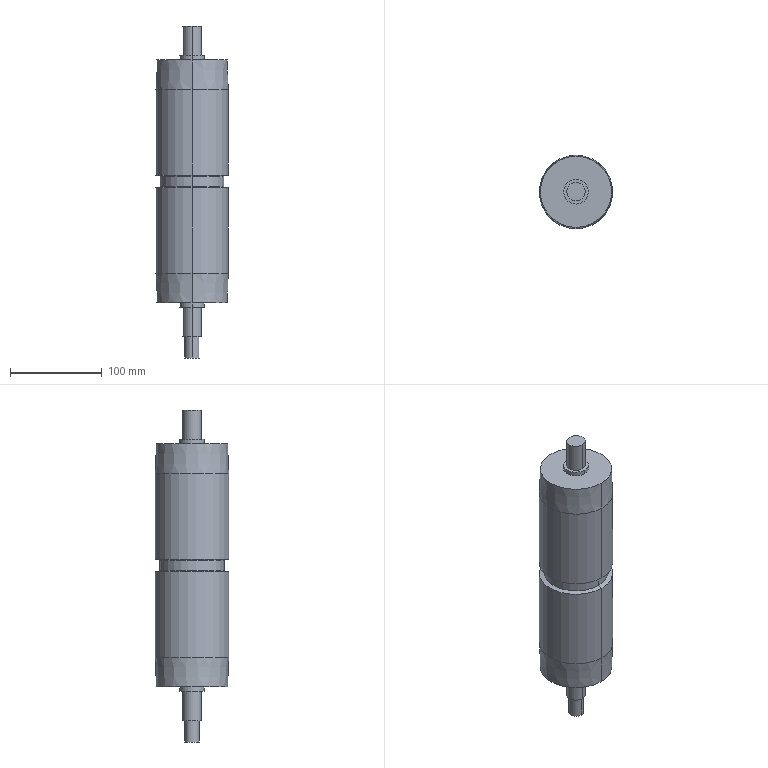Component | SolidWorks | Q1-A12-S21-Q1A.SLDASQ-1_Q1-A12-S21-Q1A-03A-1 | 1 solid | 31 faces | box 80 x 80 x 362.1 mm | volume 1338088 mm3 | cylinder 16 | cone 8 | plane 7 | commonest cylinder face diameters 27 x4 20 x4 80 x4 16 x2 70 x2 | material SUJ2
build123d program:
from build123d import *

# Parameters (mm, degrees)
SKETCH2_R           = 8
BOSS_EXTRUDE1_DEPTH = 23


with BuildPart() as part:
    # Sketch1 → Revolve1 (revolve)
    with BuildSketch(Plane.XY, mode=Mode.PRIVATE) as revolve1_sk:
        Polygon((-132.5, 40), (132.5, 40), (132.5, 13.5), (137.45, 13.5), (137.45, 10), (169.55, 10), (169.55, 0), (-169.55, 0), (-169.55, 10), (-137.45, 10), (-137.45, 13.5), (-132.5, 13.5), align=None)
    revolve(revolve1_sk.sketch.rotate(Axis((-250, 0, 0), (1, 0, 0)), 180), axis=Axis((-250, 0, 0), (1, 0, 0)))

    # Sketch2 → Boss-Extrude1 (add)
    with BuildSketch(Plane.ZY.offset(169.55)):
        with Locations(Location((0, 0, 0), (0, 0, 90))):
            Circle(SKETCH2_R)
    extrude(amount=BOSS_EXTRUDE1_DEPTH)

    # Sketch4 → Cut-Revolve1 (revolve, cut)
    with BuildSketch(Plane.XY):
        Polygon((-7, 40), (-5.9, 35), (5.9, 35), (7, 40), align=None)
    revolve(axis=Axis((-250, 0, 0), (-1, 0, 0)), mode=Mode.SUBTRACT)

    # Sketch5 → Cut-Revolve2 (revolve, cut)
    with BuildSketch(Plane.XY):
        Polygon((-132.5, 38.865), (-100, 40), (-132.5, 40), align=None)
        Polygon((132.5, 40), (100, 40), (132.5, 38.865), align=None)
    revolve(axis=Axis((-250, 0, 0), (-1, 0, 0)), mode=Mode.SUBTRACT)


solid = part.part

# Placed as in the assembly
solid = solid.moved(Location((0, 0, 0), (0, -90, 0)))
STEP:
#1=COLOUR_RGB('',0.7922,0.8196,0.9333);
#2=FILL_AREA_STYLE_COLOUR('',#1);
#3=FILL_AREA_STYLE('',(#2));
#4=SURFACE_STYLE_FILL_AREA(#3);
#5=SURFACE_SIDE_STYLE('',(#4));
#6=SURFACE_STYLE_USAGE(.BOTH.,#5);
#7=PRESENTATION_STYLE_ASSIGNMENT((#6));
#8=CARTESIAN_POINT('',(0.,-0.5315,5.411));
#9=VERTEX_POINT('',#8);
#10=CARTESIAN_POINT('',(0.,0.5315,5.411));
#11=VERTEX_POINT('',#10);
#12=CARTESIAN_POINT('',(0.,0.,5.411));
#13=DIRECTION('',(-0.,-0.,-1.));
#14=DIRECTION('',(0.,-1.,0.));
#15=AXIS2_PLACEMENT_3D('',#12,#13,#14);
#16=CIRCLE('',#15,0.5315);
#17=EDGE_CURVE('',#9,#11,#16,.T.);
#18=ORIENTED_EDGE('',*,*,#17,.T.);
#19=CARTESIAN_POINT('',(0.,0.5315,5.217));
#20=VERTEX_POINT('',#19);
#21=CARTESIAN_POINT('',(-0.,0.5315,-9.843));
#22=DIRECTION('',(-0.,-0.,-1.));
#23=VECTOR('',#22,39.37);
#24=LINE('',#21,#23);
#25=EDGE_CURVE('',#11,#20,#24,.T.);
#26=ORIENTED_EDGE('',*,*,#25,.T.);
#27=CARTESIAN_POINT('',(0.,-0.5315,5.217));
#28=VERTEX_POINT('',#27);
#29=CARTESIAN_POINT('',(0.,0.,5.217));
#30=DIRECTION('',(-0.,-0.,-1.));
#31=DIRECTION('',(0.,-1.,0.));
#32=AXIS2_PLACEMENT_3D('',#29,#30,#31);
#33=CIRCLE('',#32,0.5315);
#34=EDGE_CURVE('',#28,#20,#33,.T.);
#35=ORIENTED_EDGE('',*,*,#34,.F.);
#36=CARTESIAN_POINT('',(-0.,-0.5315,-9.843));
#37=DIRECTION('',(-0.,-0.,-1.));
#38=VECTOR('',#37,39.37);
#39=LINE('',#36,#38);
#40=EDGE_CURVE('',#9,#28,#39,.T.);
#41=ORIENTED_EDGE('',*,*,#40,.F.);
#42=EDGE_LOOP('',(#18,#26,#35,#41));
#43=FACE_OUTER_BOUND('',#42,.T.);
#44=CARTESIAN_POINT('',(-0.,0.,-9.843));
#45=DIRECTION('',(-0.,-0.,-1.));
#46=DIRECTION('',(0.,-1.,0.));
#47=AXIS2_PLACEMENT_3D('',#44,#45,#46);
#48=CYLINDRICAL_SURFACE('',#47,0.5315);
#49=ADVANCED_FACE('',(#43),#48,.T.);
#50=CARTESIAN_POINT('',(0.,-0.3937,6.675));
#51=VERTEX_POINT('',#50);
#52=CARTESIAN_POINT('',(0.,0.3937,6.675));
#53=VERTEX_POINT('',#52);
#54=CARTESIAN_POINT('',(0.,0.,6.675));
#55=DIRECTION('',(-0.,-0.,-1.));
#56=DIRECTION('',(0.,-1.,0.));
#57=AXIS2_PLACEMENT_3D('',#54,#55,#56);
#58=CIRCLE('',#57,0.3937);
#59=EDGE_CURVE('',#51,#53,#58,.T.);
#60=ORIENTED_EDGE('',*,*,#59,.T.);
#61=CARTESIAN_POINT('',(0.,0.3937,5.411));
#62=VERTEX_POINT('',#61);
#63=CARTESIAN_POINT('',(-0.,0.3937,-9.843));
#64=DIRECTION('',(-0.,-0.,-1.));
#65=VECTOR('',#64,39.37);
#66=LINE('',#63,#65);
#67=EDGE_CURVE('',#53,#62,#66,.T.);
#68=ORIENTED_EDGE('',*,*,#67,.T.);
#69=CARTESIAN_POINT('',(0.,-0.3937,5.411));
#70=VERTEX_POINT('',#69);
#71=CARTESIAN_POINT('',(0.,0.,5.411));
#72=DIRECTION('',(-0.,-0.,-1.));
#73=DIRECTION('',(0.,-1.,0.));
#74=AXIS2_PLACEMENT_3D('',#71,#72,#73);
#75=CIRCLE('',#74,0.3937);
#76=EDGE_CURVE('',#70,#62,#75,.T.);
#77=ORIENTED_EDGE('',*,*,#76,.F.);
#78=CARTESIAN_POINT('',(-0.,-0.3937,-9.843));
#79=DIRECTION('',(-0.,-0.,-1.));
#80=VECTOR('',#79,39.37);
#81=LINE('',#78,#80);
#82=EDGE_CURVE('',#51,#70,#81,.T.);
#83=ORIENTED_EDGE('',*,*,#82,.F.);
#84=EDGE_LOOP('',(#60,#68,#77,#83));
#85=FACE_OUTER_BOUND('',#84,.T.);
#86=CARTESIAN_POINT('',(-0.,0.,-9.843));
#87=DIRECTION('',(-0.,-0.,-1.));
#88=DIRECTION('',(0.,-1.,0.));
#89=AXIS2_PLACEMENT_3D('',#86,#87,#88);
#90=CYLINDRICAL_SURFACE('',#89,0.3937);
#91=ADVANCED_FACE('',(#85),#90,.T.);
#92=CARTESIAN_POINT('',(-0.,1.53,5.217));
#93=VERTEX_POINT('',#92);
#94=CARTESIAN_POINT('',(0.,-1.53,5.217));
#95=VERTEX_POINT('',#94);
#96=CARTESIAN_POINT('',(0.,0.,5.217));
#97=DIRECTION('',(0.,0.,1.));
#98=DIRECTION('',(-0.,1.,0.));
#99=AXIS2_PLACEMENT_3D('',#96,#97,#98);
#100=CIRCLE('',#99,1.53);
#101=EDGE_CURVE('',#93,#95,#100,.T.);
#102=ORIENTED_EDGE('',*,*,#101,.F.);
#103=CARTESIAN_POINT('',(-0.,1.575,3.937));
#104=VERTEX_POINT('',#103);
#105=CARTESIAN_POINT('',(-0.,1.575,3.937));
#106=DIRECTION('',(-0.,0.0349,-0.9994));
#107=VECTOR('',#106,39.37);
#108=LINE('',#105,#107);
#109=EDGE_CURVE('',#93,#104,#108,.T.);
#110=ORIENTED_EDGE('',*,*,#109,.T.);
#111=CARTESIAN_POINT('',(0.,-1.575,3.937));
#112=VERTEX_POINT('',#111);
#113=CARTESIAN_POINT('',(0.,0.,3.937));
#114=DIRECTION('',(0.,0.,1.));
#115=DIRECTION('',(-0.,1.,0.));
#116=AXIS2_PLACEMENT_3D('',#113,#114,#115);
#117=CIRCLE('',#116,1.575);
#118=EDGE_CURVE('',#104,#112,#117,.T.);
#119=ORIENTED_EDGE('',*,*,#118,.T.);
#120=CARTESIAN_POINT('',(0.,-1.575,3.937));
#121=DIRECTION('',(-0.,-0.0349,-0.9994));
#122=VECTOR('',#121,39.37);
#123=LINE('',#120,#122);
#124=EDGE_CURVE('',#95,#112,#123,.T.);
#125=ORIENTED_EDGE('',*,*,#124,.F.);
#126=EDGE_LOOP('',(#102,#110,#119,#125));
#127=FACE_OUTER_BOUND('',#126,.T.);
#128=CARTESIAN_POINT('',(0.,0.,3.937));
#129=DIRECTION('',(-0.,-0.,-1.));
#130=DIRECTION('',(0.,-1.,0.));
#131=AXIS2_PLACEMENT_3D('',#128,#129,#130);
#132=CONICAL_SURFACE('',#131,1.575,0.03491);
#133=ADVANCED_FACE('',(#127),#132,.T.);
#134=CARTESIAN_POINT('',(-0.,-0.5315,-5.217));
#135=VERTEX_POINT('',#134);
#136=CARTESIAN_POINT('',(-0.,0.5315,-5.217));
#137=VERTEX_POINT('',#136);
#138=CARTESIAN_POINT('',(-0.,0.,-5.217));
#139=DIRECTION('',(-0.,-0.,-1.));
#140=DIRECTION('',(0.,-1.,0.));
#141=AXIS2_PLACEMENT_3D('',#138,#139,#140);
#142=CIRCLE('',#141,0.5315);
#143=EDGE_CURVE('',#135,#137,#142,.T.);
#144=ORIENTED_EDGE('',*,*,#143,.T.);
#145=CARTESIAN_POINT('',(-0.,0.5315,-5.411));
#146=VERTEX_POINT('',#145);
#147=CARTESIAN_POINT('',(-0.,0.5315,-9.843));
#148=DIRECTION('',(-0.,-0.,-1.));
#149=VECTOR('',#148,39.37);
#150=LINE('',#147,#149);
#151=EDGE_CURVE('',#137,#146,#150,.T.);
#152=ORIENTED_EDGE('',*,*,#151,.T.);
#153=CARTESIAN_POINT('',(-0.,-0.5315,-5.411));
#154=VERTEX_POINT('',#153);
#155=CARTESIAN_POINT('',(-0.,0.,-5.411));
#156=DIRECTION('',(-0.,-0.,-1.));
#157=DIRECTION('',(0.,-1.,0.));
#158=AXIS2_PLACEMENT_3D('',#155,#156,#157);
#159=CIRCLE('',#158,0.5315);
#160=EDGE_CURVE('',#154,#146,#159,.T.);
#161=ORIENTED_EDGE('',*,*,#160,.F.);
#162=CARTESIAN_POINT('',(-0.,-0.5315,-9.843));
#163=DIRECTION('',(-0.,-0.,-1.));
#164=VECTOR('',#163,39.37);
#165=LINE('',#162,#164);
#166=EDGE_CURVE('',#135,#154,#165,.T.);
#167=ORIENTED_EDGE('',*,*,#166,.F.);
#168=EDGE_LOOP('',(#144,#152,#161,#167));
#169=FACE_OUTER_BOUND('',#168,.T.);
#170=CARTESIAN_POINT('',(-0.,0.,-9.843));
#171=DIRECTION('',(-0.,-0.,-1.));
#172=DIRECTION('',(0.,-1.,0.));
#173=AXIS2_PLACEMENT_3D('',#170,#171,#172);
#174=CYLINDRICAL_SURFACE('',#173,0.5315);
#175=ADVANCED_FACE('',(#169),#174,.T.);
#176=CARTESIAN_POINT('',(-0.,-0.3937,-5.411));
#177=VERTEX_POINT('',#176);
#178=CARTESIAN_POINT('',(-0.,0.3937,-5.411));
#179=VERTEX_POINT('',#178);
#180=CARTESIAN_POINT('',(-0.,0.,-5.411));
#181=DIRECTION('',(-0.,-0.,-1.));
#182=DIRECTION('',(0.,-1.,0.));
#183=AXIS2_PLACEMENT_3D('',#180,#181,#182);
#184=CIRCLE('',#183,0.3937);
#185=EDGE_CURVE('',#177,#179,#184,.T.);
#186=ORIENTED_EDGE('',*,*,#185,.T.);
#187=CARTESIAN_POINT('',(-0.,0.3937,-6.675));
#188=VERTEX_POINT('',#187);
#189=CARTESIAN_POINT('',(-0.,0.3937,-9.843));
#190=DIRECTION('',(-0.,-0.,-1.));
#191=VECTOR('',#190,39.37);
#192=LINE('',#189,#191);
#193=EDGE_CURVE('',#179,#188,#192,.T.);
#194=ORIENTED_EDGE('',*,*,#193,.T.);
#195=CARTESIAN_POINT('',(-0.,-0.3937,-6.675));
#196=VERTEX_POINT('',#195);
#197=CARTESIAN_POINT('',(-0.,0.,-6.675));
#198=DIRECTION('',(-0.,-0.,-1.));
#199=DIRECTION('',(0.,-1.,0.));
#200=AXIS2_PLACEMENT_3D('',#197,#198,#199);
#201=CIRCLE('',#200,0.3937);
#202=EDGE_CURVE('',#196,#188,#201,.T.);
#203=ORIENTED_EDGE('',*,*,#202,.F.);
#204=CARTESIAN_POINT('',(-0.,-0.3937,-9.843));
#205=DIRECTION('',(-0.,-0.,-1.));
#206=VECTOR('',#205,39.37);
#207=LINE('',#204,#206);
#208=EDGE_CURVE('',#177,#196,#207,.T.);
#209=ORIENTED_EDGE('',*,*,#208,.F.);
#210=EDGE_LOOP('',(#186,#194,#203,#209));
#211=FACE_OUTER_BOUND('',#210,.T.);
#212=CARTESIAN_POINT('',(-0.,0.,-9.843));
#213=DIRECTION('',(-0.,-0.,-1.));
#214=DIRECTION('',(0.,-1.,0.));
#215=AXIS2_PLACEMENT_3D('',#212,#213,#214);
#216=CYLINDRICAL_SURFACE('',#215,0.3937);
#217=ADVANCED_FACE('',(#211),#216,.T.);
#218=CARTESIAN_POINT('',(-0.,-0.315,-7.581));
#219=VERTEX_POINT('',#218);
#220=CARTESIAN_POINT('',(-0.,0.315,-7.581));
#221=VERTEX_POINT('',#220);
#222=CARTESIAN_POINT('',(-0.,0.,-7.581));
#223=DIRECTION('',(-0.,-0.,-1.));
#224=DIRECTION('',(0.,-1.,0.));
#225=AXIS2_PLACEMENT_3D('',#222,#223,#224);
#226=CIRCLE('',#225,0.315);
#227=EDGE_CURVE('',#219,#221,#226,.T.);
#228=ORIENTED_EDGE('',*,*,#227,.F.);
#229=CARTESIAN_POINT('',(-0.,-0.315,-6.675));
#230=VERTEX_POINT('',#229);
#231=CARTESIAN_POINT('',(-0.,-0.315,-7.581));
#232=DIRECTION('',(0.,0.,1.));
#233=VECTOR('',#232,39.37);
#234=LINE('',#231,#233);
#235=EDGE_CURVE('',#219,#230,#234,.T.);
#236=ORIENTED_EDGE('',*,*,#235,.T.);
#237=CARTESIAN_POINT('',(-0.,0.315,-6.675));
#238=VERTEX_POINT('',#237);
#239=CARTESIAN_POINT('',(-0.,0.,-6.675));
#240=DIRECTION('',(-0.,-0.,-1.));
#241=DIRECTION('',(-0.,1.,0.));
#242=AXIS2_PLACEMENT_3D('',#239,#240,#241);
#243=CIRCLE('',#242,0.315);
#244=EDGE_CURVE('',#230,#238,#243,.T.);
#245=ORIENTED_EDGE('',*,*,#244,.T.);
#246=CARTESIAN_POINT('',(-0.,0.315,-7.581));
#247=DIRECTION('',(0.,0.,1.));
#248=VECTOR('',#247,39.37);
#249=LINE('',#246,#248);
#250=EDGE_CURVE('',#221,#238,#249,.T.);
#251=ORIENTED_EDGE('',*,*,#250,.F.);
#252=EDGE_LOOP('',(#228,#236,#245,#251));
#253=FACE_OUTER_BOUND('',#252,.T.);
#254=CARTESIAN_POINT('',(-0.,0.,-7.581));
#255=DIRECTION('',(0.,0.,1.));
#256=DIRECTION('',(-0.,1.,0.));
#257=AXIS2_PLACEMENT_3D('',#254,#255,#256);
#258=CYLINDRICAL_SURFACE('',#257,0.315);
#259=ADVANCED_FACE('',(#253),#258,.T.);
#260=CARTESIAN_POINT('',(-0.,1.53,-5.217));
#261=VERTEX_POINT('',#260);
#262=CARTESIAN_POINT('',(-0.,-1.53,-5.217));
#263=VERTEX_POINT('',#262);
#264=CARTESIAN_POINT('',(-0.,0.,-5.217));
#265=DIRECTION('',(0.,0.,1.));
#266=DIRECTION('',(-0.,1.,0.));
#267=AXIS2_PLACEMENT_3D('',#264,#265,#266);
#268=CIRCLE('',#267,1.53);
#269=EDGE_CURVE('',#261,#263,#268,.T.);
#270=ORIENTED_EDGE('',*,*,#269,.T.);
#271=CARTESIAN_POINT('',(0.,-1.575,-3.937));
#272=VERTEX_POINT('',#271);
#273=CARTESIAN_POINT('',(-0.,-1.53,-5.217));
#274=DIRECTION('',(0.,-0.0349,0.9994));
#275=VECTOR('',#274,39.37);
#276=LINE('',#273,#275);
#277=EDGE_CURVE('',#263,#272,#276,.T.);
#278=ORIENTED_EDGE('',*,*,#277,.T.);
#279=CARTESIAN_POINT('',(-0.,1.575,-3.937));
#280=VERTEX_POINT('',#279);
#281=CARTESIAN_POINT('',(-0.,0.,-3.937));
#282=DIRECTION('',(0.,0.,1.));
#283=DIRECTION('',(-0.,1.,0.));
#284=AXIS2_PLACEMENT_3D('',#281,#282,#283);
#285=CIRCLE('',#284,1.575);
#286=EDGE_CURVE('',#280,#272,#285,.T.);
#287=ORIENTED_EDGE('',*,*,#286,.F.);
#288=CARTESIAN_POINT('',(-0.,1.53,-5.217));
#289=DIRECTION('',(0.,0.0349,0.9994));
#290=VECTOR('',#289,39.37);
#291=LINE('',#288,#290);
#292=EDGE_CURVE('',#261,#280,#291,.T.);
#293=ORIENTED_EDGE('',*,*,#292,.F.);
#294=EDGE_LOOP('',(#270,#278,#287,#293));
#295=FACE_OUTER_BOUND('',#294,.T.);
#296=CARTESIAN_POINT('',(-0.,0.,-5.217));
#297=DIRECTION('',(0.,0.,1.));
#298=DIRECTION('',(-0.,1.,0.));
#299=AXIS2_PLACEMENT_3D('',#296,#297,#298);
#300=CONICAL_SURFACE('',#299,1.53,0.03491);
#301=ADVANCED_FACE('',(#295),#300,.T.);
#302=ORIENTED_EDGE('',*,*,#118,.F.);
#303=CARTESIAN_POINT('',(-0.,1.575,0.2756));
#304=VERTEX_POINT('',#303);
#305=CARTESIAN_POINT('',(-0.,1.575,-9.843));
#306=DIRECTION('',(-0.,-0.,-1.));
#307=VECTOR('',#306,39.37);
#308=LINE('',#305,#307);
#309=EDGE_CURVE('',#104,#304,#308,.T.);
#310=ORIENTED_EDGE('',*,*,#309,.T.);
#311=CARTESIAN_POINT('',(-0.,-1.575,0.2756));
#312=VERTEX_POINT('',#311);
#313=CARTESIAN_POINT('',(0.,0.,0.2756));
#314=DIRECTION('',(0.,0.,1.));
#315=DIRECTION('',(-0.,1.,-0.));
#316=AXIS2_PLACEMENT_3D('',#313,#314,#315);
#317=CIRCLE('',#316,1.575);
#318=EDGE_CURVE('',#304,#312,#317,.T.);
#319=ORIENTED_EDGE('',*,*,#318,.T.);
#320=CARTESIAN_POINT('',(-0.,-1.575,-9.843));
#321=DIRECTION('',(-0.,-0.,-1.));
#322=VECTOR('',#321,39.37);
#323=LINE('',#320,#322);
#324=EDGE_CURVE('',#112,#312,#323,.T.);
#325=ORIENTED_EDGE('',*,*,#324,.F.);
#326=EDGE_LOOP('',(#302,#310,#319,#325));
#327=FACE_OUTER_BOUND('',#326,.T.);
#328=CARTESIAN_POINT('',(-0.,0.,-9.843));
#329=DIRECTION('',(-0.,-0.,-1.));
#330=DIRECTION('',(0.,-1.,0.));
#331=AXIS2_PLACEMENT_3D('',#328,#329,#330);
#332=CYLINDRICAL_SURFACE('',#331,1.575);
#333=ADVANCED_FACE('',(#327),#332,.T.);
#334=CARTESIAN_POINT('',(-0.,1.378,0.2323));
#335=VERTEX_POINT('',#334);
#336=CARTESIAN_POINT('',(-0.,-1.378,0.2323));
#337=VERTEX_POINT('',#336);
#338=CARTESIAN_POINT('',(0.,0.,0.2323));
#339=DIRECTION('',(0.,0.,1.));
#340=DIRECTION('',(-0.,1.,-0.));
#341=AXIS2_PLACEMENT_3D('',#338,#339,#340);
#342=CIRCLE('',#341,1.378);
#343=EDGE_CURVE('',#335,#337,#342,.T.);
#344=ORIENTED_EDGE('',*,*,#343,.T.);
#345=CARTESIAN_POINT('',(-0.,-1.378,0.2323));
#346=DIRECTION('',(-0.,-0.9766,0.2149));
#347=VECTOR('',#346,39.37);
#348=LINE('',#345,#347);
#349=EDGE_CURVE('',#337,#312,#348,.T.);
#350=ORIENTED_EDGE('',*,*,#349,.T.);
#351=ORIENTED_EDGE('',*,*,#318,.F.);
#352=CARTESIAN_POINT('',(-0.,1.378,0.2323));
#353=DIRECTION('',(-0.,0.9766,0.2149));
#354=VECTOR('',#353,39.37);
#355=LINE('',#352,#354);
#356=EDGE_CURVE('',#335,#304,#355,.T.);
#357=ORIENTED_EDGE('',*,*,#356,.F.);
#358=EDGE_LOOP('',(#344,#350,#351,#357));
#359=FACE_OUTER_BOUND('',#358,.T.);
#360=CARTESIAN_POINT('',(0.,0.,0.2323));
#361=DIRECTION('',(0.,0.,1.));
#362=DIRECTION('',(-0.,1.,-0.));
#363=AXIS2_PLACEMENT_3D('',#360,#361,#362);
#364=CONICAL_SURFACE('',#363,1.378,1.354);
#365=ADVANCED_FACE('',(#359),#364,.T.);
#366=CARTESIAN_POINT('',(-0.,1.378,-0.2323));
#367=VERTEX_POINT('',#366);
#368=CARTESIAN_POINT('',(0.,-1.378,-0.2323));
#369=VERTEX_POINT('',#368);
#370=CARTESIAN_POINT('',(-0.,0.,-0.2323));
#371=DIRECTION('',(0.,0.,1.));
#372=DIRECTION('',(-0.,1.,-0.));
#373=AXIS2_PLACEMENT_3D('',#370,#371,#372);
#374=CIRCLE('',#373,1.378);
#375=EDGE_CURVE('',#367,#369,#374,.T.);
#376=ORIENTED_EDGE('',*,*,#375,.T.);
#377=CARTESIAN_POINT('',(-0.,-1.378,5.217));
#378=DIRECTION('',(0.,0.,1.));
#379=VECTOR('',#378,39.37);
#380=LINE('',#377,#379);
#381=EDGE_CURVE('',#369,#337,#380,.T.);
#382=ORIENTED_EDGE('',*,*,#381,.T.);
#383=ORIENTED_EDGE('',*,*,#343,.F.);
#384=CARTESIAN_POINT('',(0.,1.378,5.217));
#385=DIRECTION('',(0.,0.,1.));
#386=VECTOR('',#385,39.37);
#387=LINE('',#384,#386);
#388=EDGE_CURVE('',#367,#335,#387,.T.);
#389=ORIENTED_EDGE('',*,*,#388,.F.);
#390=EDGE_LOOP('',(#376,#382,#383,#389));
#391=FACE_OUTER_BOUND('',#390,.T.);
#392=CARTESIAN_POINT('',(0.,0.,5.217));
#393=DIRECTION('',(0.,0.,1.));
#394=DIRECTION('',(-0.,1.,0.));
#395=AXIS2_PLACEMENT_3D('',#392,#393,#394);
#396=CYLINDRICAL_SURFACE('',#395,1.378);
#397=ADVANCED_FACE('',(#391),#396,.T.);
#398=ORIENTED_EDGE('',*,*,#375,.F.);
#399=CARTESIAN_POINT('',(-0.,1.575,-0.2756));
#400=VERTEX_POINT('',#399);
#401=CARTESIAN_POINT('',(-0.,1.575,-0.2756));
#402=DIRECTION('',(-0.,0.9766,-0.2149));
#403=VECTOR('',#402,39.37);
#404=LINE('',#401,#403);
#405=EDGE_CURVE('',#367,#400,#404,.T.);
#406=ORIENTED_EDGE('',*,*,#405,.T.);
#407=CARTESIAN_POINT('',(0.,-1.575,-0.2756));
#408=VERTEX_POINT('',#407);
#409=CARTESIAN_POINT('',(-0.,0.,-0.2756));
#410=DIRECTION('',(0.,0.,1.));
#411=DIRECTION('',(-0.,1.,-0.));
#412=AXIS2_PLACEMENT_3D('',#409,#410,#411);
#413=CIRCLE('',#412,1.575);
#414=EDGE_CURVE('',#400,#408,#413,.T.);
#415=ORIENTED_EDGE('',*,*,#414,.T.);
#416=CARTESIAN_POINT('',(0.,-1.575,-0.2756));
#417=DIRECTION('',(0.,-0.9766,-0.2149));
#418=VECTOR('',#417,39.37);
#419=LINE('',#416,#418);
#420=EDGE_CURVE('',#369,#408,#419,.T.);
#421=ORIENTED_EDGE('',*,*,#420,.F.);
#422=EDGE_LOOP('',(#398,#406,#415,#421));
#423=FACE_OUTER_BOUND('',#422,.T.);
#424=CARTESIAN_POINT('',(-0.,0.,-0.2756));
#425=DIRECTION('',(-0.,-0.,-1.));
#426=DIRECTION('',(0.,-1.,0.));
#427=AXIS2_PLACEMENT_3D('',#424,#425,#426);
#428=CONICAL_SURFACE('',#427,1.575,1.354);
#429=ADVANCED_FACE('',(#423),#428,.T.);
#430=ORIENTED_EDGE('',*,*,#414,.F.);
#431=CARTESIAN_POINT('',(-0.,1.575,-9.843));
#432=DIRECTION('',(-0.,-0.,-1.));
#433=VECTOR('',#432,39.37);
#434=LINE('',#431,#433);
#435=EDGE_CURVE('',#400,#280,#434,.T.);
#436=ORIENTED_EDGE('',*,*,#435,.T.);
#437=ORIENTED_EDGE('',*,*,#286,.T.);
#438=CARTESIAN_POINT('',(-0.,-1.575,-9.843));
#439=DIRECTION('',(-0.,-0.,-1.));
#440=VECTOR('',#439,39.37);
#441=LINE('',#438,#440);
#442=EDGE_CURVE('',#408,#272,#441,.T.);
#443=ORIENTED_EDGE('',*,*,#442,.F.);
#444=EDGE_LOOP('',(#430,#436,#437,#443));
#445=FACE_OUTER_BOUND('',#444,.T.);
#446=CARTESIAN_POINT('',(-0.,0.,-9.843));
#447=DIRECTION('',(-0.,-0.,-1.));
#448=DIRECTION('',(0.,-1.,0.));
#449=AXIS2_PLACEMENT_3D('',#446,#447,#448);
#450=CYLINDRICAL_SURFACE('',#449,1.575);
#451=ADVANCED_FACE('',(#445),#450,.T.);
#452=ORIENTED_EDGE('',*,*,#435,.F.);
#453=CARTESIAN_POINT('',(-0.,0.,-0.2756));
#454=DIRECTION('',(0.,0.,1.));
#455=DIRECTION('',(-0.,1.,-0.));
#456=AXIS2_PLACEMENT_3D('',#453,#454,#455);
#457=CIRCLE('',#456,1.575);
#458=EDGE_CURVE('',#408,#400,#457,.T.);
#459=ORIENTED_EDGE('',*,*,#458,.F.);
#460=ORIENTED_EDGE('',*,*,#442,.T.);
#461=CARTESIAN_POINT('',(-0.,0.,-3.937));
#462=DIRECTION('',(0.,0.,1.));
#463=DIRECTION('',(-0.,1.,0.));
#464=AXIS2_PLACEMENT_3D('',#461,#462,#463);
#465=CIRCLE('',#464,1.575);
#466=EDGE_CURVE('',#272,#280,#465,.T.);
#467=ORIENTED_EDGE('',*,*,#466,.T.);
#468=EDGE_LOOP('',(#452,#459,#460,#467));
#469=FACE_OUTER_BOUND('',#468,.T.);
#470=CARTESIAN_POINT('',(-0.,0.,-9.843));
#471=DIRECTION('',(-0.,-0.,-1.));
#472=DIRECTION('',(0.,-1.,0.));
#473=AXIS2_PLACEMENT_3D('',#470,#471,#472);
#474=CYLINDRICAL_SURFACE('',#473,1.575);
#475=ADVANCED_FACE('',(#469),#474,.T.);
#476=ORIENTED_EDGE('',*,*,#405,.F.);
#477=CARTESIAN_POINT('',(-0.,0.,-0.2323));
#478=DIRECTION('',(0.,0.,1.));
#479=DIRECTION('',(-0.,1.,-0.));
#480=AXIS2_PLACEMENT_3D('',#477,#478,#479);
#481=CIRCLE('',#480,1.378);
#482=EDGE_CURVE('',#369,#367,#481,.T.);
#483=ORIENTED_EDGE('',*,*,#482,.F.);
#484=ORIENTED_EDGE('',*,*,#420,.T.);
#485=ORIENTED_EDGE('',*,*,#458,.T.);
#486=EDGE_LOOP('',(#476,#483,#484,#485));
#487=FACE_OUTER_BOUND('',#486,.T.);
#488=CARTESIAN_POINT('',(-0.,0.,-0.2756));
#489=DIRECTION('',(-0.,-0.,-1.));
#490=DIRECTION('',(0.,-1.,0.));
#491=AXIS2_PLACEMENT_3D('',#488,#489,#490);
#492=CONICAL_SURFACE('',#491,1.575,1.354);
#493=ADVANCED_FACE('',(#487),#492,.T.);
#494=ORIENTED_EDGE('',*,*,#381,.F.);
#495=ORIENTED_EDGE('',*,*,#482,.T.);
#496=ORIENTED_EDGE('',*,*,#388,.T.);
#497=CARTESIAN_POINT('',(0.,0.,0.2323));
#498=DIRECTION('',(0.,0.,1.));
#499=DIRECTION('',(-0.,1.,-0.));
#500=AXIS2_PLACEMENT_3D('',#497,#498,#499);
#501=CIRCLE('',#500,1.378);
#502=EDGE_CURVE('',#337,#335,#501,.T.);
#503=ORIENTED_EDGE('',*,*,#502,.F.);
#504=EDGE_LOOP('',(#494,#495,#496,#503));
#505=FACE_OUTER_BOUND('',#504,.T.);
#506=CARTESIAN_POINT('',(0.,0.,5.217));
#507=DIRECTION('',(0.,0.,1.));
#508=DIRECTION('',(-0.,1.,0.));
#509=AXIS2_PLACEMENT_3D('',#506,#507,#508);
#510=CYLINDRICAL_SURFACE('',#509,1.378);
#511=ADVANCED_FACE('',(#505),#510,.T.);
#512=ORIENTED_EDGE('',*,*,#349,.F.);
#513=ORIENTED_EDGE('',*,*,#502,.T.);
#514=ORIENTED_EDGE('',*,*,#356,.T.);
#515=CARTESIAN_POINT('',(0.,0.,0.2756));
#516=DIRECTION('',(0.,0.,1.));
#517=DIRECTION('',(-0.,1.,-0.));
#518=AXIS2_PLACEMENT_3D('',#515,#516,#517);
#519=CIRCLE('',#518,1.575);
#520=EDGE_CURVE('',#312,#304,#519,.T.);
#521=ORIENTED_EDGE('',*,*,#520,.F.);
#522=EDGE_LOOP('',(#512,#513,#514,#521));
#523=FACE_OUTER_BOUND('',#522,.T.);
#524=CARTESIAN_POINT('',(0.,0.,0.2323));
#525=DIRECTION('',(0.,0.,1.));
#526=DIRECTION('',(-0.,1.,-0.));
#527=AXIS2_PLACEMENT_3D('',#524,#525,#526);
#528=CONICAL_SURFACE('',#527,1.378,1.354);
#529=ADVANCED_FACE('',(#523),#528,.T.);
#530=ORIENTED_EDGE('',*,*,#309,.F.);
#531=CARTESIAN_POINT('',(0.,0.,3.937));
#532=DIRECTION('',(0.,0.,1.));
#533=DIRECTION('',(-0.,1.,0.));
#534=AXIS2_PLACEMENT_3D('',#531,#532,#533);
#535=CIRCLE('',#534,1.575);
#536=EDGE_CURVE('',#112,#104,#535,.T.);
#537=ORIENTED_EDGE('',*,*,#536,.F.);
#538=ORIENTED_EDGE('',*,*,#324,.T.);
#539=ORIENTED_EDGE('',*,*,#520,.T.);
#540=EDGE_LOOP('',(#530,#537,#538,#539));
#541=FACE_OUTER_BOUND('',#540,.T.);
#542=CARTESIAN_POINT('',(-0.,0.,-9.843));
#543=DIRECTION('',(-0.,-0.,-1.));
#544=DIRECTION('',(0.,-1.,0.));
#545=AXIS2_PLACEMENT_3D('',#542,#543,#544);
#546=CYLINDRICAL_SURFACE('',#545,1.575);
#547=ADVANCED_FACE('',(#541),#546,.T.);
#548=ORIENTED_EDGE('',*,*,#277,.F.);
#549=CARTESIAN_POINT('',(-0.,0.,-5.217));
#550=DIRECTION('',(0.,0.,1.));
#551=DIRECTION('',(-0.,1.,0.));
#552=AXIS2_PLACEMENT_3D('',#549,#550,#551);
#553=CIRCLE('',#552,1.53);
#554=EDGE_CURVE('',#263,#261,#553,.T.);
#555=ORIENTED_EDGE('',*,*,#554,.T.);
#556=ORIENTED_EDGE('',*,*,#292,.T.);
#557=ORIENTED_EDGE('',*,*,#466,.F.);
#558=EDGE_LOOP('',(#548,#555,#556,#557));
#559=FACE_OUTER_BOUND('',#558,.T.);
#560=CARTESIAN_POINT('',(-0.,0.,-5.217));
#561=DIRECTION('',(0.,0.,1.));
#562=DIRECTION('',(-0.,1.,0.));
#563=AXIS2_PLACEMENT_3D('',#560,#561,#562);
#564=CONICAL_SURFACE('',#563,1.53,0.03491);
#565=ADVANCED_FACE('',(#559),#564,.T.);
#566=CARTESIAN_POINT('',(-0.,0.,-7.581));
#567=DIRECTION('',(-0.,-0.,-1.));
#568=DIRECTION('',(0.,-1.,0.));
#569=AXIS2_PLACEMENT_3D('',#566,#567,#568);
#570=CIRCLE('',#569,0.315);
#571=EDGE_CURVE('',#221,#219,#570,.T.);
#572=ORIENTED_EDGE('',*,*,#571,.T.);
#573=ORIENTED_EDGE('',*,*,#227,.T.);
#574=EDGE_LOOP('',(#572,#573));
#575=FACE_OUTER_BOUND('',#574,.T.);
#576=CARTESIAN_POINT('',(-0.,0.,-7.581));
#577=DIRECTION('',(-0.,-0.,-1.));
#578=DIRECTION('',(0.,-1.,0.));
#579=AXIS2_PLACEMENT_3D('',#576,#577,#578);
#580=PLANE('',#579);
#581=ADVANCED_FACE('',(#575),#580,.T.);
#582=ORIENTED_EDGE('',*,*,#235,.F.);
#583=ORIENTED_EDGE('',*,*,#571,.F.);
#584=ORIENTED_EDGE('',*,*,#250,.T.);
#585=CARTESIAN_POINT('',(-0.,0.,-6.675));
#586=DIRECTION('',(-0.,-0.,-1.));
#587=DIRECTION('',(-0.,1.,0.));
#588=AXIS2_PLACEMENT_3D('',#585,#586,#587);
#589=CIRCLE('',#588,0.315);
#590=EDGE_CURVE('',#238,#230,#589,.T.);
#591=ORIENTED_EDGE('',*,*,#590,.T.);
#592=EDGE_LOOP('',(#582,#583,#584,#591));
#593=FACE_OUTER_BOUND('',#592,.T.);
#594=CARTESIAN_POINT('',(-0.,0.,-7.581));
#595=DIRECTION('',(0.,0.,1.));
#596=DIRECTION('',(-0.,1.,0.));
#597=AXIS2_PLACEMENT_3D('',#594,#595,#596);
#598=CYLINDRICAL_SURFACE('',#597,0.315);
#599=ADVANCED_FACE('',(#593),#598,.T.);
#600=ORIENTED_EDGE('',*,*,#590,.F.);
#601=ORIENTED_EDGE('',*,*,#244,.F.);
#602=EDGE_LOOP('',(#600,#601));
#603=FACE_BOUND('',#602,.T.);
#604=ORIENTED_EDGE('',*,*,#202,.T.);
#605=CARTESIAN_POINT('',(-0.,0.,-6.675));
#606=DIRECTION('',(-0.,-0.,-1.));
#607=DIRECTION('',(0.,-1.,0.));
#608=AXIS2_PLACEMENT_3D('',#605,#606,#607);
#609=CIRCLE('',#608,0.3937);
#610=EDGE_CURVE('',#188,#196,#609,.T.);
#611=ORIENTED_EDGE('',*,*,#610,.T.);
#612=EDGE_LOOP('',(#604,#611));
#613=FACE_OUTER_BOUND('',#612,.T.);
#614=CARTESIAN_POINT('',(-0.,0.3937,-6.675));
#615=DIRECTION('',(0.,0.,1.));
#616=DIRECTION('',(-0.,1.,-0.));
#617=AXIS2_PLACEMENT_3D('',#614,#615,#616);
#618=PLANE('',#617);
#619=ADVANCED_FACE('',(#603,#613),#618,.F.);
#620=ORIENTED_EDGE('',*,*,#193,.F.);
#621=CARTESIAN_POINT('',(-0.,0.,-5.411));
#622=DIRECTION('',(-0.,-0.,-1.));
#623=DIRECTION('',(0.,-1.,0.));
#624=AXIS2_PLACEMENT_3D('',#621,#622,#623);
#625=CIRCLE('',#624,0.3937);
#626=EDGE_CURVE('',#179,#177,#625,.T.);
#627=ORIENTED_EDGE('',*,*,#626,.T.);
#628=ORIENTED_EDGE('',*,*,#208,.T.);
#629=ORIENTED_EDGE('',*,*,#610,.F.);
#630=EDGE_LOOP('',(#620,#627,#628,#629));
#631=FACE_OUTER_BOUND('',#630,.T.);
#632=CARTESIAN_POINT('',(-0.,0.,-9.843));
#633=DIRECTION('',(-0.,-0.,-1.));
#634=DIRECTION('',(0.,-1.,0.));
#635=AXIS2_PLACEMENT_3D('',#632,#633,#634);
#636=CYLINDRICAL_SURFACE('',#635,0.3937);
#637=ADVANCED_FACE('',(#631),#636,.T.);
#638=ORIENTED_EDGE('',*,*,#185,.F.);
#639=ORIENTED_EDGE('',*,*,#626,.F.);
#640=EDGE_LOOP('',(#638,#639));
#641=FACE_BOUND('',#640,.T.);
#642=ORIENTED_EDGE('',*,*,#160,.T.);
#643=CARTESIAN_POINT('',(-0.,0.,-5.411));
#644=DIRECTION('',(-0.,-0.,-1.));
#645=DIRECTION('',(0.,-1.,0.));
#646=AXIS2_PLACEMENT_3D('',#643,#644,#645);
#647=CIRCLE('',#646,0.5315);
#648=EDGE_CURVE('',#146,#154,#647,.T.);
#649=ORIENTED_EDGE('',*,*,#648,.T.);
#650=EDGE_LOOP('',(#642,#649));
#651=FACE_OUTER_BOUND('',#650,.T.);
#652=CARTESIAN_POINT('',(-0.,0.5315,-5.411));
#653=DIRECTION('',(0.,0.,1.));
#654=DIRECTION('',(-0.,1.,-0.));
#655=AXIS2_PLACEMENT_3D('',#652,#653,#654);
#656=PLANE('',#655);
#657=ADVANCED_FACE('',(#641,#651),#656,.F.);
#658=ORIENTED_EDGE('',*,*,#151,.F.);
#659=CARTESIAN_POINT('',(-0.,0.,-5.217));
#660=DIRECTION('',(-0.,-0.,-1.));
#661=DIRECTION('',(0.,-1.,0.));
#662=AXIS2_PLACEMENT_3D('',#659,#660,#661);
#663=CIRCLE('',#662,0.5315);
#664=EDGE_CURVE('',#137,#135,#663,.T.);
#665=ORIENTED_EDGE('',*,*,#664,.T.);
#666=ORIENTED_EDGE('',*,*,#166,.T.);
#667=ORIENTED_EDGE('',*,*,#648,.F.);
#668=EDGE_LOOP('',(#658,#665,#666,#667));
#669=FACE_OUTER_BOUND('',#668,.T.);
#670=CARTESIAN_POINT('',(-0.,0.,-9.843));
#671=DIRECTION('',(-0.,-0.,-1.));
#672=DIRECTION('',(0.,-1.,0.));
#673=AXIS2_PLACEMENT_3D('',#670,#671,#672);
#674=CYLINDRICAL_SURFACE('',#673,0.5315);
#675=ADVANCED_FACE('',(#669),#674,.T.);
#676=ORIENTED_EDGE('',*,*,#143,.F.);
#677=ORIENTED_EDGE('',*,*,#664,.F.);
#678=EDGE_LOOP('',(#676,#677));
#679=FACE_BOUND('',#678,.T.);
#680=ORIENTED_EDGE('',*,*,#269,.F.);
#681=ORIENTED_EDGE('',*,*,#554,.F.);
#682=EDGE_LOOP('',(#680,#681));
#683=FACE_OUTER_BOUND('',#682,.T.);
#684=CARTESIAN_POINT('',(-0.,0.5315,-5.217));
#685=DIRECTION('',(0.,0.,1.));
#686=DIRECTION('',(-0.,1.,-0.));
#687=AXIS2_PLACEMENT_3D('',#684,#685,#686);
#688=PLANE('',#687);
#689=ADVANCED_FACE('',(#679,#683),#688,.F.);
#690=ORIENTED_EDGE('',*,*,#109,.F.);
#691=CARTESIAN_POINT('',(0.,0.,5.217));
#692=DIRECTION('',(0.,0.,1.));
#693=DIRECTION('',(-0.,1.,0.));
#694=AXIS2_PLACEMENT_3D('',#691,#692,#693);
#695=CIRCLE('',#694,1.53);
#696=EDGE_CURVE('',#95,#93,#695,.T.);
#697=ORIENTED_EDGE('',*,*,#696,.F.);
#698=ORIENTED_EDGE('',*,*,#124,.T.);
#699=ORIENTED_EDGE('',*,*,#536,.T.);
#700=EDGE_LOOP('',(#690,#697,#698,#699));
#701=FACE_OUTER_BOUND('',#700,.T.);
#702=CARTESIAN_POINT('',(0.,0.,3.937));
#703=DIRECTION('',(-0.,-0.,-1.));
#704=DIRECTION('',(0.,-1.,0.));
#705=AXIS2_PLACEMENT_3D('',#702,#703,#704);
#706=CONICAL_SURFACE('',#705,1.575,0.03491);
#707=ADVANCED_FACE('',(#701),#706,.T.);
#708=ORIENTED_EDGE('',*,*,#59,.F.);
#709=CARTESIAN_POINT('',(0.,0.,6.675));
#710=DIRECTION('',(-0.,-0.,-1.));
#711=DIRECTION('',(0.,-1.,0.));
#712=AXIS2_PLACEMENT_3D('',#709,#710,#711);
#713=CIRCLE('',#712,0.3937);
#714=EDGE_CURVE('',#53,#51,#713,.T.);
#715=ORIENTED_EDGE('',*,*,#714,.F.);
#716=EDGE_LOOP('',(#708,#715));
#717=FACE_OUTER_BOUND('',#716,.T.);
#718=CARTESIAN_POINT('',(0.,0.3937,6.675));
#719=DIRECTION('',(-0.,-0.,-1.));
#720=DIRECTION('',(0.,-1.,0.));
#721=AXIS2_PLACEMENT_3D('',#718,#719,#720);
#722=PLANE('',#721);
#723=ADVANCED_FACE('',(#717),#722,.F.);
#724=ORIENTED_EDGE('',*,*,#67,.F.);
#725=ORIENTED_EDGE('',*,*,#714,.T.);
#726=ORIENTED_EDGE('',*,*,#82,.T.);
#727=CARTESIAN_POINT('',(0.,0.,5.411));
#728=DIRECTION('',(-0.,-0.,-1.));
#729=DIRECTION('',(0.,-1.,0.));
#730=AXIS2_PLACEMENT_3D('',#727,#728,#729);
#731=CIRCLE('',#730,0.3937);
#732=EDGE_CURVE('',#62,#70,#731,.T.);
#733=ORIENTED_EDGE('',*,*,#732,.F.);
#734=EDGE_LOOP('',(#724,#725,#726,#733));
#735=FACE_OUTER_BOUND('',#734,.T.);
#736=CARTESIAN_POINT('',(-0.,0.,-9.843));
#737=DIRECTION('',(-0.,-0.,-1.));
#738=DIRECTION('',(0.,-1.,0.));
#739=AXIS2_PLACEMENT_3D('',#736,#737,#738);
#740=CYLINDRICAL_SURFACE('',#739,0.3937);
#741=ADVANCED_FACE('',(#735),#740,.T.);
#742=ORIENTED_EDGE('',*,*,#17,.F.);
#743=CARTESIAN_POINT('',(0.,0.,5.411));
#744=DIRECTION('',(-0.,-0.,-1.));
#745=DIRECTION('',(0.,-1.,0.));
#746=AXIS2_PLACEMENT_3D('',#743,#744,#745);
#747=CIRCLE('',#746,0.5315);
#748=EDGE_CURVE('',#11,#9,#747,.T.);
#749=ORIENTED_EDGE('',*,*,#748,.F.);
#750=EDGE_LOOP('',(#742,#749));
#751=FACE_OUTER_BOUND('',#750,.T.);
#752=ORIENTED_EDGE('',*,*,#76,.T.);
#753=ORIENTED_EDGE('',*,*,#732,.T.);
#754=EDGE_LOOP('',(#752,#753));
#755=FACE_BOUND('',#754,.T.);
#756=CARTESIAN_POINT('',(0.,0.5315,5.411));
#757=DIRECTION('',(-0.,-0.,-1.));
#758=DIRECTION('',(0.,-1.,0.));
#759=AXIS2_PLACEMENT_3D('',#756,#757,#758);
#760=PLANE('',#759);
#761=ADVANCED_FACE('',(#751,#755),#760,.F.);
#762=ORIENTED_EDGE('',*,*,#25,.F.);
#763=ORIENTED_EDGE('',*,*,#748,.T.);
#764=ORIENTED_EDGE('',*,*,#40,.T.);
#765=CARTESIAN_POINT('',(0.,0.,5.217));
#766=DIRECTION('',(-0.,-0.,-1.));
#767=DIRECTION('',(0.,-1.,0.));
#768=AXIS2_PLACEMENT_3D('',#765,#766,#767);
#769=CIRCLE('',#768,0.5315);
#770=EDGE_CURVE('',#20,#28,#769,.T.);
#771=ORIENTED_EDGE('',*,*,#770,.F.);
#772=EDGE_LOOP('',(#762,#763,#764,#771));
#773=FACE_OUTER_BOUND('',#772,.T.);
#774=CARTESIAN_POINT('',(-0.,0.,-9.843));
#775=DIRECTION('',(-0.,-0.,-1.));
#776=DIRECTION('',(0.,-1.,0.));
#777=AXIS2_PLACEMENT_3D('',#774,#775,#776);
#778=CYLINDRICAL_SURFACE('',#777,0.5315);
#779=ADVANCED_FACE('',(#773),#778,.T.);
#780=ORIENTED_EDGE('',*,*,#34,.T.);
#781=ORIENTED_EDGE('',*,*,#770,.T.);
#782=EDGE_LOOP('',(#780,#781));
#783=FACE_BOUND('',#782,.T.);
#784=ORIENTED_EDGE('',*,*,#696,.T.);
#785=ORIENTED_EDGE('',*,*,#101,.T.);
#786=EDGE_LOOP('',(#784,#785));
#787=FACE_OUTER_BOUND('',#786,.T.);
#788=CARTESIAN_POINT('',(0.,1.575,5.217));
#789=DIRECTION('',(-0.,-0.,-1.));
#790=DIRECTION('',(0.,-1.,0.));
#791=AXIS2_PLACEMENT_3D('',#788,#789,#790);
#792=PLANE('',#791);
#793=ADVANCED_FACE('',(#783,#787),#792,.F.);
#794=CLOSED_SHELL('',(#49,#91,#133,#175,#217,#259,#301,#333,#365,#397,#429,#451,#475,#493,#511,#529,#547,#565,#581,#599,#619,#637,#657,#675,#689,#707,#723,#741,#761,#779,#793));
#795=MANIFOLD_SOLID_BREP('',#794);
#796=STYLED_ITEM('',(#7),#795);
#797=PRESENTATION_LAYER_ASSIGNMENT('','',(#796));
#798=(LENGTH_UNIT()NAMED_UNIT(*)SI_UNIT($,.METRE.));
#799=LENGTH_MEASURE_WITH_UNIT(LENGTH_MEASURE(0.0254),#798);
#800=DIMENSIONAL_EXPONENTS(1.,0.,0.,0.,0.,0.,0.);
#801=(CONVERSION_BASED_UNIT('',#799)LENGTH_UNIT()NAMED_UNIT(#800));
#802=UNCERTAINTY_MEASURE_WITH_UNIT(LENGTH_MEASURE(0.00001),#801,'','');
#803=(NAMED_UNIT(*)PLANE_ANGLE_UNIT()SI_UNIT($,.RADIAN.));
#804=(NAMED_UNIT(*)SI_UNIT($,.STERADIAN.)SOLID_ANGLE_UNIT());
#805=(GEOMETRIC_REPRESENTATION_CONTEXT(3)GLOBAL_UNCERTAINTY_ASSIGNED_CONTEXT((#802))GLOBAL_UNIT_ASSIGNED_CONTEXT((#801,#803,#804))REPRESENTATION_CONTEXT('',''));
#806=MECHANICAL_DESIGN_GEOMETRIC_PRESENTATION_REPRESENTATION('',(#796),#805);
#807=CARTESIAN_POINT('',(0.,0.,0.));
#808=DIRECTION('',(0.,0.,1.));
#809=DIRECTION('',(1.,0.,0.));
#810=AXIS2_PLACEMENT_3D('',#807,#808,#809);
#811=(LENGTH_UNIT()NAMED_UNIT(*)SI_UNIT($,.METRE.));
#812=LENGTH_MEASURE_WITH_UNIT(LENGTH_MEASURE(0.0254),#811);
#813=DIMENSIONAL_EXPONENTS(1.,0.,0.,0.,0.,0.,0.);
#814=(CONVERSION_BASED_UNIT('',#812)LENGTH_UNIT()NAMED_UNIT(#813));
#815=UNCERTAINTY_MEASURE_WITH_UNIT(LENGTH_MEASURE(0.00001),#814,'','');
#816=(NAMED_UNIT(*)PLANE_ANGLE_UNIT()SI_UNIT($,.RADIAN.));
#817=(NAMED_UNIT(*)SI_UNIT($,.STERADIAN.)SOLID_ANGLE_UNIT());
#818=(GEOMETRIC_REPRESENTATION_CONTEXT(3)GLOBAL_UNCERTAINTY_ASSIGNED_CONTEXT((#815))GLOBAL_UNIT_ASSIGNED_CONTEXT((#814,#816,#817))REPRESENTATION_CONTEXT('',''));
#819=ADVANCED_BREP_SHAPE_REPRESENTATION('',(#795,#810),#818);